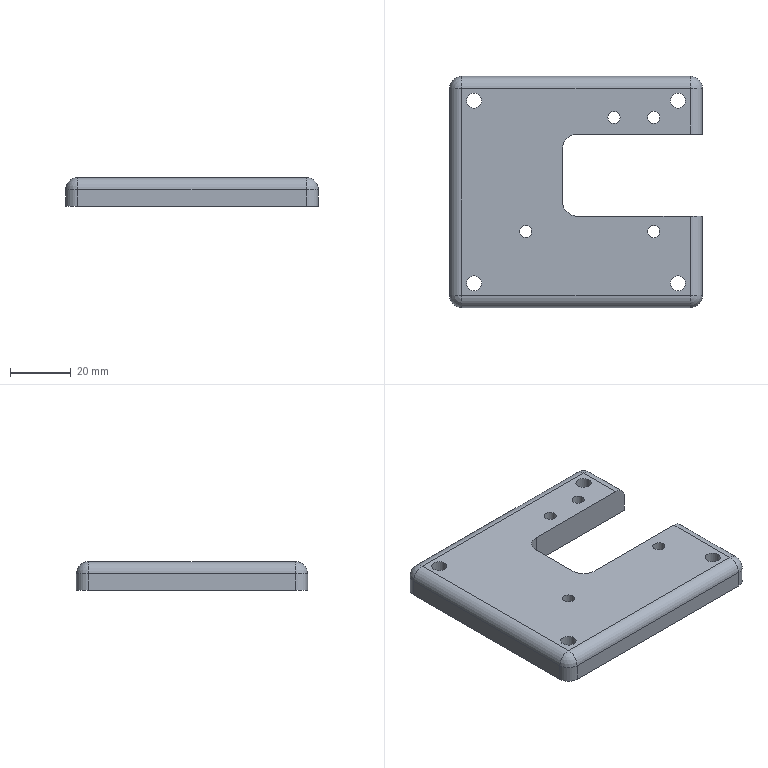Component | NX | BASE_PLATE | 1 solid | 37 faces | volume 45912 mm3 | cylinder 19 | plane 10 | sphere 4 | cone 4 | commonest cylinder face diameters 8 x9 5 x4 4 x4 10 x2